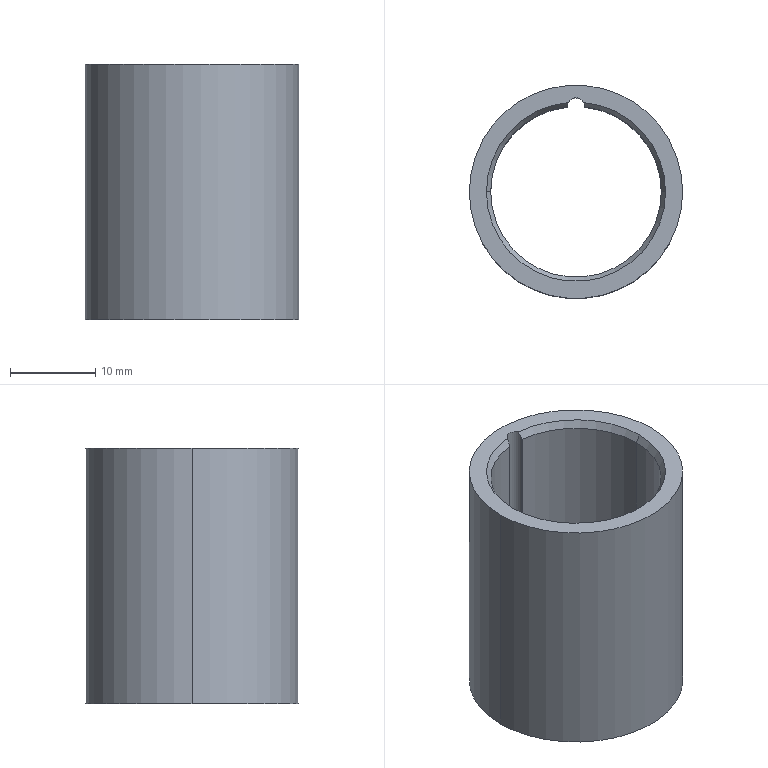Component | SolidWorks | Bushing-1 | 1 solid | 13 faces | box 25 x 25 x 30 mm | volume 5240 mm3 | cylinder 8 | cone 3 | plane 2 | commonest cylinder face diameters 2 x3 20 x3 25 x2
STEP:
#1=CARTESIAN_POINT('',(-3.217,-0.7278,5.906));
#2=VERTEX_POINT('',#1);
#3=CARTESIAN_POINT('',(-3.217,-0.7297,5.906));
#4=VERTEX_POINT('',#3);
#5=CARTESIAN_POINT('',(-3.178,-0.7278,5.906));
#6=DIRECTION('',(0.,0.,1.));
#7=DIRECTION('',(1.,0.,0.));
#8=AXIS2_PLACEMENT_3D('',#5,#6,#7);
#9=CIRCLE('',#8,0.03937);
#10=EDGE_CURVE('',#2,#4,#9,.T.);
#11=ORIENTED_EDGE('',*,*,#10,.F.);
#12=CARTESIAN_POINT('',(-3.217,-0.7278,7.056));
#13=VERTEX_POINT('',#12);
#14=CARTESIAN_POINT('',(-3.217,-0.7278,5.551));
#15=DIRECTION('',(0.,0.,1.));
#16=VECTOR('',#15,39.37);
#17=LINE('',#14,#16);
#18=EDGE_CURVE('',#2,#13,#17,.T.);
#19=ORIENTED_EDGE('',*,*,#18,.T.);
#20=CARTESIAN_POINT('',(-3.217,-0.7297,7.053));
#21=VERTEX_POINT('',#20);
#22=CARTESIAN_POINT('',(-3.217,-0.7278,7.056));
#23=CARTESIAN_POINT('',(-3.217,-0.7284,7.055));
#24=CARTESIAN_POINT('',(-3.217,-0.7291,7.054));
#25=CARTESIAN_POINT('',(-3.217,-0.7297,7.053));
#26=B_SPLINE_CURVE_WITH_KNOTS('',3,(#22,#23,#24,#25),.UNSPECIFIED.,.F.,.F.,(4,4),(0.0009137,0.001013),.UNSPECIFIED.);
#27=EDGE_CURVE('',#13,#21,#26,.T.);
#28=ORIENTED_EDGE('',*,*,#27,.T.);
#29=CARTESIAN_POINT('',(-3.217,-0.7297,7.087));
#30=DIRECTION('',(0.,0.,-1.));
#31=VECTOR('',#30,39.37);
#32=LINE('',#29,#31);
#33=EDGE_CURVE('',#21,#4,#32,.T.);
#34=ORIENTED_EDGE('',*,*,#33,.T.);
#35=EDGE_LOOP('',(#11,#19,#28,#34));
#36=FACE_OUTER_BOUND('',#35,.T.);
#37=CARTESIAN_POINT('',(-3.178,-0.7278,5.551));
#38=DIRECTION('',(0.,0.,1.));
#39=DIRECTION('',(1.,0.,0.));
#40=AXIS2_PLACEMENT_3D('',#37,#38,#39);
#41=CYLINDRICAL_SURFACE('',#40,0.03937);
#42=ADVANCED_FACE('',(#36),#41,.F.);
#43=ORIENTED_EDGE('',*,*,#18,.F.);
#44=CARTESIAN_POINT('',(-3.139,-0.7278,5.906));
#45=VERTEX_POINT('',#44);
#46=CARTESIAN_POINT('',(-3.178,-0.7278,5.906));
#47=DIRECTION('',(0.,0.,1.));
#48=DIRECTION('',(1.,0.,0.));
#49=AXIS2_PLACEMENT_3D('',#46,#47,#48);
#50=CIRCLE('',#49,0.03937);
#51=EDGE_CURVE('',#45,#2,#50,.T.);
#52=ORIENTED_EDGE('',*,*,#51,.F.);
#53=CARTESIAN_POINT('',(-3.139,-0.7278,7.056));
#54=VERTEX_POINT('',#53);
#55=CARTESIAN_POINT('',(-3.139,-0.7278,5.551));
#56=DIRECTION('',(0.,0.,1.));
#57=VECTOR('',#56,39.37);
#58=LINE('',#55,#57);
#59=EDGE_CURVE('',#45,#54,#58,.T.);
#60=ORIENTED_EDGE('',*,*,#59,.T.);
#61=CARTESIAN_POINT('',(-3.143,-0.7096,7.087));
#62=VERTEX_POINT('',#61);
#63=CARTESIAN_POINT('',(-3.139,-0.7278,7.056));
#64=CARTESIAN_POINT('',(-3.139,-0.7217,7.066));
#65=CARTESIAN_POINT('',(-3.14,-0.7156,7.077));
#66=CARTESIAN_POINT('',(-3.143,-0.7096,7.087));
#67=B_SPLINE_CURVE_WITH_KNOTS('',3,(#63,#64,#65,#66),.UNSPECIFIED.,.F.,.F.,(4,4),(0.00009929,0.001013),.UNSPECIFIED.);
#68=EDGE_CURVE('',#54,#62,#67,.T.);
#69=ORIENTED_EDGE('',*,*,#68,.T.);
#70=CARTESIAN_POINT('',(-3.213,-0.7096,7.087));
#71=VERTEX_POINT('',#70);
#72=CARTESIAN_POINT('',(-3.178,-0.7278,7.087));
#73=DIRECTION('',(0.,0.,1.));
#74=DIRECTION('',(1.,0.,0.));
#75=AXIS2_PLACEMENT_3D('',#72,#73,#74);
#76=CIRCLE('',#75,0.03937);
#77=EDGE_CURVE('',#62,#71,#76,.T.);
#78=ORIENTED_EDGE('',*,*,#77,.T.);
#79=CARTESIAN_POINT('',(-3.213,-0.7096,7.087));
#80=CARTESIAN_POINT('',(-3.216,-0.7156,7.077));
#81=CARTESIAN_POINT('',(-3.217,-0.7217,7.066));
#82=CARTESIAN_POINT('',(-3.217,-0.7278,7.056));
#83=B_SPLINE_CURVE_WITH_KNOTS('',3,(#79,#80,#81,#82),.UNSPECIFIED.,.F.,.F.,(4,4),(0.00000024,0.0009137),.UNSPECIFIED.);
#84=EDGE_CURVE('',#71,#13,#83,.T.);
#85=ORIENTED_EDGE('',*,*,#84,.T.);
#86=EDGE_LOOP('',(#43,#52,#60,#69,#78,#85));
#87=FACE_OUTER_BOUND('',#86,.T.);
#88=CARTESIAN_POINT('',(-3.178,-0.7278,5.551));
#89=DIRECTION('',(0.,0.,1.));
#90=DIRECTION('',(1.,0.,0.));
#91=AXIS2_PLACEMENT_3D('',#88,#89,#90);
#92=CYLINDRICAL_SURFACE('',#91,0.03937);
#93=ADVANCED_FACE('',(#87),#92,.F.);
#94=CARTESIAN_POINT('',(-3.572,-1.121,7.053));
#95=VERTEX_POINT('',#94);
#96=CARTESIAN_POINT('',(-2.784,-1.121,7.053));
#97=VERTEX_POINT('',#96);
#98=CARTESIAN_POINT('',(-3.178,-1.121,7.053));
#99=DIRECTION('',(0.,0.,1.));
#100=DIRECTION('',(1.,0.,0.));
#101=AXIS2_PLACEMENT_3D('',#98,#99,#100);
#102=CIRCLE('',#101,0.3937);
#103=EDGE_CURVE('',#95,#97,#102,.T.);
#104=ORIENTED_EDGE('',*,*,#103,.F.);
#105=CARTESIAN_POINT('',(-3.591,-1.121,7.087));
#106=VERTEX_POINT('',#105);
#107=CARTESIAN_POINT('',(-3.572,-1.121,7.053));
#108=DIRECTION('',(-0.5,0.,0.866));
#109=VECTOR('',#108,39.37);
#110=LINE('',#107,#109);
#111=EDGE_CURVE('',#95,#106,#110,.T.);
#112=ORIENTED_EDGE('',*,*,#111,.T.);
#113=CARTESIAN_POINT('',(-2.765,-1.121,7.087));
#114=VERTEX_POINT('',#113);
#115=CARTESIAN_POINT('',(-3.178,-1.121,7.087));
#116=DIRECTION('',(0.,0.,-1.));
#117=DIRECTION('',(1.,0.,0.));
#118=AXIS2_PLACEMENT_3D('',#115,#116,#117);
#119=CIRCLE('',#118,0.4134);
#120=EDGE_CURVE('',#114,#106,#119,.T.);
#121=ORIENTED_EDGE('',*,*,#120,.F.);
#122=CARTESIAN_POINT('',(-2.784,-1.121,7.053));
#123=DIRECTION('',(0.5,0.,0.866));
#124=VECTOR('',#123,39.37);
#125=LINE('',#122,#124);
#126=EDGE_CURVE('',#97,#114,#125,.T.);
#127=ORIENTED_EDGE('',*,*,#126,.F.);
#128=EDGE_LOOP('',(#104,#112,#121,#127));
#129=FACE_OUTER_BOUND('',#128,.T.);
#130=CARTESIAN_POINT('',(-3.178,-1.121,7.053));
#131=DIRECTION('',(0.,0.,1.));
#132=DIRECTION('',(1.,0.,0.));
#133=AXIS2_PLACEMENT_3D('',#130,#131,#132);
#134=CONICAL_SURFACE('',#133,0.3937,0.5236);
#135=ADVANCED_FACE('',(#129),#134,.F.);
#136=CARTESIAN_POINT('',(-3.139,-0.7297,7.053));
#137=VERTEX_POINT('',#136);
#138=CARTESIAN_POINT('',(-3.178,-1.121,7.053));
#139=DIRECTION('',(0.,0.,1.));
#140=DIRECTION('',(1.,0.,0.));
#141=AXIS2_PLACEMENT_3D('',#138,#139,#140);
#142=CIRCLE('',#141,0.3937);
#143=EDGE_CURVE('',#97,#137,#142,.T.);
#144=ORIENTED_EDGE('',*,*,#143,.F.);
#145=ORIENTED_EDGE('',*,*,#126,.T.);
#146=CARTESIAN_POINT('',(-3.178,-1.121,7.087));
#147=DIRECTION('',(0.,0.,-1.));
#148=DIRECTION('',(1.,-0.,0.));
#149=AXIS2_PLACEMENT_3D('',#146,#147,#148);
#150=CIRCLE('',#149,0.4134);
#151=EDGE_CURVE('',#62,#114,#150,.T.);
#152=ORIENTED_EDGE('',*,*,#151,.F.);
#153=ORIENTED_EDGE('',*,*,#68,.F.);
#154=CARTESIAN_POINT('',(-3.139,-0.7297,7.053));
#155=CARTESIAN_POINT('',(-3.139,-0.7291,7.054));
#156=CARTESIAN_POINT('',(-3.139,-0.7284,7.055));
#157=CARTESIAN_POINT('',(-3.139,-0.7278,7.056));
#158=B_SPLINE_CURVE_WITH_KNOTS('',3,(#154,#155,#156,#157),.UNSPECIFIED.,.F.,.F.,(4,4),(0.00000023,0.00009929),.UNSPECIFIED.);
#159=EDGE_CURVE('',#137,#54,#158,.T.);
#160=ORIENTED_EDGE('',*,*,#159,.F.);
#161=EDGE_LOOP('',(#144,#145,#152,#153,#160));
#162=FACE_OUTER_BOUND('',#161,.T.);
#163=CARTESIAN_POINT('',(-3.178,-1.121,7.053));
#164=DIRECTION('',(0.,0.,1.));
#165=DIRECTION('',(1.,0.,0.));
#166=AXIS2_PLACEMENT_3D('',#163,#164,#165);
#167=CONICAL_SURFACE('',#166,0.3937,0.5236);
#168=ADVANCED_FACE('',(#162),#167,.F.);
#169=ORIENTED_EDGE('',*,*,#103,.T.);
#170=CARTESIAN_POINT('',(-2.784,-1.121,5.906));
#171=VERTEX_POINT('',#170);
#172=CARTESIAN_POINT('',(-2.784,-1.121,7.087));
#173=DIRECTION('',(0.,0.,-1.));
#174=VECTOR('',#173,39.37);
#175=LINE('',#172,#174);
#176=EDGE_CURVE('',#97,#171,#175,.T.);
#177=ORIENTED_EDGE('',*,*,#176,.T.);
#178=CARTESIAN_POINT('',(-3.572,-1.121,5.906));
#179=VERTEX_POINT('',#178);
#180=CARTESIAN_POINT('',(-3.178,-1.121,5.906));
#181=DIRECTION('',(0.,0.,1.));
#182=DIRECTION('',(1.,0.,0.));
#183=AXIS2_PLACEMENT_3D('',#180,#181,#182);
#184=CIRCLE('',#183,0.3937);
#185=EDGE_CURVE('',#179,#171,#184,.T.);
#186=ORIENTED_EDGE('',*,*,#185,.F.);
#187=CARTESIAN_POINT('',(-3.572,-1.121,7.087));
#188=DIRECTION('',(0.,0.,-1.));
#189=VECTOR('',#188,39.37);
#190=LINE('',#187,#189);
#191=EDGE_CURVE('',#95,#179,#190,.T.);
#192=ORIENTED_EDGE('',*,*,#191,.F.);
#193=EDGE_LOOP('',(#169,#177,#186,#192));
#194=FACE_OUTER_BOUND('',#193,.T.);
#195=CARTESIAN_POINT('',(-3.178,-1.121,7.087));
#196=DIRECTION('',(0.,0.,-1.));
#197=DIRECTION('',(-1.,0.,0.));
#198=AXIS2_PLACEMENT_3D('',#195,#196,#197);
#199=CYLINDRICAL_SURFACE('',#198,0.3937);
#200=ADVANCED_FACE('',(#194),#199,.F.);
#201=CARTESIAN_POINT('',(-3.178,-1.121,7.053));
#202=DIRECTION('',(0.,0.,1.));
#203=DIRECTION('',(1.,0.,0.));
#204=AXIS2_PLACEMENT_3D('',#201,#202,#203);
#205=CIRCLE('',#204,0.3937);
#206=EDGE_CURVE('',#21,#95,#205,.T.);
#207=ORIENTED_EDGE('',*,*,#206,.T.);
#208=ORIENTED_EDGE('',*,*,#191,.T.);
#209=CARTESIAN_POINT('',(-3.178,-1.121,5.906));
#210=DIRECTION('',(0.,0.,1.));
#211=DIRECTION('',(1.,0.,0.));
#212=AXIS2_PLACEMENT_3D('',#209,#210,#211);
#213=CIRCLE('',#212,0.3937);
#214=EDGE_CURVE('',#4,#179,#213,.T.);
#215=ORIENTED_EDGE('',*,*,#214,.F.);
#216=ORIENTED_EDGE('',*,*,#33,.F.);
#217=EDGE_LOOP('',(#207,#208,#215,#216));
#218=FACE_OUTER_BOUND('',#217,.T.);
#219=CARTESIAN_POINT('',(-3.178,-1.121,7.087));
#220=DIRECTION('',(0.,0.,-1.));
#221=DIRECTION('',(-1.,0.,0.));
#222=AXIS2_PLACEMENT_3D('',#219,#220,#221);
#223=CYLINDRICAL_SURFACE('',#222,0.3937);
#224=ADVANCED_FACE('',(#218),#223,.F.);
#225=CARTESIAN_POINT('',(-2.686,-1.121,7.087));
#226=VERTEX_POINT('',#225);
#227=CARTESIAN_POINT('',(-3.67,-1.121,7.087));
#228=VERTEX_POINT('',#227);
#229=CARTESIAN_POINT('',(-3.178,-1.121,7.087));
#230=DIRECTION('',(0.,0.,1.));
#231=DIRECTION('',(1.,0.,0.));
#232=AXIS2_PLACEMENT_3D('',#229,#230,#231);
#233=CIRCLE('',#232,0.4921);
#234=EDGE_CURVE('',#226,#228,#233,.T.);
#235=ORIENTED_EDGE('',*,*,#234,.F.);
#236=CARTESIAN_POINT('',(-2.686,-1.121,5.906));
#237=VERTEX_POINT('',#236);
#238=CARTESIAN_POINT('',(-2.686,-1.121,7.087));
#239=DIRECTION('',(0.,0.,-1.));
#240=VECTOR('',#239,39.37);
#241=LINE('',#238,#240);
#242=EDGE_CURVE('',#226,#237,#241,.T.);
#243=ORIENTED_EDGE('',*,*,#242,.T.);
#244=CARTESIAN_POINT('',(-3.67,-1.121,5.906));
#245=VERTEX_POINT('',#244);
#246=CARTESIAN_POINT('',(-3.178,-1.121,5.906));
#247=DIRECTION('',(0.,0.,1.));
#248=DIRECTION('',(1.,0.,0.));
#249=AXIS2_PLACEMENT_3D('',#246,#247,#248);
#250=CIRCLE('',#249,0.4921);
#251=EDGE_CURVE('',#237,#245,#250,.T.);
#252=ORIENTED_EDGE('',*,*,#251,.T.);
#253=CARTESIAN_POINT('',(-3.67,-1.121,7.087));
#254=DIRECTION('',(0.,0.,-1.));
#255=VECTOR('',#254,39.37);
#256=LINE('',#253,#255);
#257=EDGE_CURVE('',#228,#245,#256,.T.);
#258=ORIENTED_EDGE('',*,*,#257,.F.);
#259=EDGE_LOOP('',(#235,#243,#252,#258));
#260=FACE_OUTER_BOUND('',#259,.T.);
#261=CARTESIAN_POINT('',(-3.178,-1.121,7.087));
#262=DIRECTION('',(0.,0.,-1.));
#263=DIRECTION('',(-1.,0.,0.));
#264=AXIS2_PLACEMENT_3D('',#261,#262,#263);
#265=CYLINDRICAL_SURFACE('',#264,0.4921);
#266=ADVANCED_FACE('',(#260),#265,.T.);
#267=ORIENTED_EDGE('',*,*,#77,.F.);
#268=ORIENTED_EDGE('',*,*,#151,.T.);
#269=ORIENTED_EDGE('',*,*,#120,.T.);
#270=CARTESIAN_POINT('',(-3.178,-1.121,7.087));
#271=DIRECTION('',(0.,0.,-1.));
#272=DIRECTION('',(1.,0.,0.));
#273=AXIS2_PLACEMENT_3D('',#270,#271,#272);
#274=CIRCLE('',#273,0.4134);
#275=EDGE_CURVE('',#106,#71,#274,.T.);
#276=ORIENTED_EDGE('',*,*,#275,.T.);
#277=EDGE_LOOP('',(#267,#268,#269,#276));
#278=FACE_BOUND('',#277,.T.);
#279=CARTESIAN_POINT('',(-3.178,-1.121,7.087));
#280=DIRECTION('',(0.,0.,1.));
#281=DIRECTION('',(1.,0.,0.));
#282=AXIS2_PLACEMENT_3D('',#279,#280,#281);
#283=CIRCLE('',#282,0.4921);
#284=EDGE_CURVE('',#228,#226,#283,.T.);
#285=ORIENTED_EDGE('',*,*,#284,.T.);
#286=ORIENTED_EDGE('',*,*,#234,.T.);
#287=EDGE_LOOP('',(#285,#286));
#288=FACE_OUTER_BOUND('',#287,.T.);
#289=CARTESIAN_POINT('',(-3.178,-1.121,7.087));
#290=DIRECTION('',(0.,0.,1.));
#291=DIRECTION('',(1.,0.,0.));
#292=AXIS2_PLACEMENT_3D('',#289,#290,#291);
#293=PLANE('',#292);
#294=ADVANCED_FACE('',(#278,#288),#293,.T.);
#295=CARTESIAN_POINT('',(-3.178,-1.121,5.906));
#296=DIRECTION('',(0.,0.,1.));
#297=DIRECTION('',(1.,0.,0.));
#298=AXIS2_PLACEMENT_3D('',#295,#296,#297);
#299=CIRCLE('',#298,0.4921);
#300=EDGE_CURVE('',#245,#237,#299,.T.);
#301=ORIENTED_EDGE('',*,*,#300,.F.);
#302=ORIENTED_EDGE('',*,*,#251,.F.);
#303=EDGE_LOOP('',(#301,#302));
#304=FACE_OUTER_BOUND('',#303,.T.);
#305=ORIENTED_EDGE('',*,*,#214,.T.);
#306=ORIENTED_EDGE('',*,*,#185,.T.);
#307=CARTESIAN_POINT('',(-3.139,-0.7297,5.906));
#308=VERTEX_POINT('',#307);
#309=CARTESIAN_POINT('',(-3.178,-1.121,5.906));
#310=DIRECTION('',(0.,0.,1.));
#311=DIRECTION('',(1.,0.,0.));
#312=AXIS2_PLACEMENT_3D('',#309,#310,#311);
#313=CIRCLE('',#312,0.3937);
#314=EDGE_CURVE('',#171,#308,#313,.T.);
#315=ORIENTED_EDGE('',*,*,#314,.T.);
#316=CARTESIAN_POINT('',(-3.178,-0.7278,5.906));
#317=DIRECTION('',(0.,0.,1.));
#318=DIRECTION('',(1.,0.,0.));
#319=AXIS2_PLACEMENT_3D('',#316,#317,#318);
#320=CIRCLE('',#319,0.03937);
#321=EDGE_CURVE('',#308,#45,#320,.T.);
#322=ORIENTED_EDGE('',*,*,#321,.T.);
#323=ORIENTED_EDGE('',*,*,#51,.T.);
#324=ORIENTED_EDGE('',*,*,#10,.T.);
#325=EDGE_LOOP('',(#305,#306,#315,#322,#323,#324));
#326=FACE_BOUND('',#325,.T.);
#327=CARTESIAN_POINT('',(-3.178,-1.121,5.906));
#328=DIRECTION('',(0.,0.,1.));
#329=DIRECTION('',(1.,0.,0.));
#330=AXIS2_PLACEMENT_3D('',#327,#328,#329);
#331=PLANE('',#330);
#332=ADVANCED_FACE('',(#304,#326),#331,.F.);
#333=ORIENTED_EDGE('',*,*,#242,.F.);
#334=ORIENTED_EDGE('',*,*,#284,.F.);
#335=ORIENTED_EDGE('',*,*,#257,.T.);
#336=ORIENTED_EDGE('',*,*,#300,.T.);
#337=EDGE_LOOP('',(#333,#334,#335,#336));
#338=FACE_OUTER_BOUND('',#337,.T.);
#339=CARTESIAN_POINT('',(-3.178,-1.121,7.087));
#340=DIRECTION('',(0.,0.,-1.));
#341=DIRECTION('',(-1.,0.,0.));
#342=AXIS2_PLACEMENT_3D('',#339,#340,#341);
#343=CYLINDRICAL_SURFACE('',#342,0.4921);
#344=ADVANCED_FACE('',(#338),#343,.T.);
#345=ORIENTED_EDGE('',*,*,#176,.F.);
#346=ORIENTED_EDGE('',*,*,#143,.T.);
#347=CARTESIAN_POINT('',(-3.139,-0.7297,7.087));
#348=DIRECTION('',(0.,0.,1.));
#349=VECTOR('',#348,39.37);
#350=LINE('',#347,#349);
#351=EDGE_CURVE('',#308,#137,#350,.T.);
#352=ORIENTED_EDGE('',*,*,#351,.F.);
#353=ORIENTED_EDGE('',*,*,#314,.F.);
#354=EDGE_LOOP('',(#345,#346,#352,#353));
#355=FACE_OUTER_BOUND('',#354,.T.);
#356=CARTESIAN_POINT('',(-3.178,-1.121,7.087));
#357=DIRECTION('',(0.,0.,-1.));
#358=DIRECTION('',(-1.,0.,0.));
#359=AXIS2_PLACEMENT_3D('',#356,#357,#358);
#360=CYLINDRICAL_SURFACE('',#359,0.3937);
#361=ADVANCED_FACE('',(#355),#360,.F.);
#362=ORIENTED_EDGE('',*,*,#111,.F.);
#363=ORIENTED_EDGE('',*,*,#206,.F.);
#364=ORIENTED_EDGE('',*,*,#27,.F.);
#365=ORIENTED_EDGE('',*,*,#84,.F.);
#366=ORIENTED_EDGE('',*,*,#275,.F.);
#367=EDGE_LOOP('',(#362,#363,#364,#365,#366));
#368=FACE_OUTER_BOUND('',#367,.T.);
#369=CARTESIAN_POINT('',(-3.178,-1.121,7.053));
#370=DIRECTION('',(0.,0.,1.));
#371=DIRECTION('',(1.,0.,0.));
#372=AXIS2_PLACEMENT_3D('',#369,#370,#371);
#373=CONICAL_SURFACE('',#372,0.3937,0.5236);
#374=ADVANCED_FACE('',(#368),#373,.F.);
#375=ORIENTED_EDGE('',*,*,#59,.F.);
#376=ORIENTED_EDGE('',*,*,#321,.F.);
#377=ORIENTED_EDGE('',*,*,#351,.T.);
#378=ORIENTED_EDGE('',*,*,#159,.T.);
#379=EDGE_LOOP('',(#375,#376,#377,#378));
#380=FACE_OUTER_BOUND('',#379,.T.);
#381=CARTESIAN_POINT('',(-3.178,-0.7278,5.551));
#382=DIRECTION('',(0.,0.,1.));
#383=DIRECTION('',(1.,0.,0.));
#384=AXIS2_PLACEMENT_3D('',#381,#382,#383);
#385=CYLINDRICAL_SURFACE('',#384,0.03937);
#386=ADVANCED_FACE('',(#380),#385,.F.);
#387=CLOSED_SHELL('',(#42,#93,#135,#168,#200,#224,#266,#294,#332,#344,#361,#374,#386));
#388=MANIFOLD_SOLID_BREP('',#387);
#389=CARTESIAN_POINT('',(0.,0.,0.));
#390=DIRECTION('',(0.,0.,1.));
#391=DIRECTION('',(1.,0.,0.));
#392=AXIS2_PLACEMENT_3D('',#389,#390,#391);
#393=(LENGTH_UNIT()NAMED_UNIT(*)SI_UNIT($,.METRE.));
#394=LENGTH_MEASURE_WITH_UNIT(LENGTH_MEASURE(0.0254),#393);
#395=DIMENSIONAL_EXPONENTS(1.,0.,0.,0.,0.,0.,0.);
#396=(CONVERSION_BASED_UNIT('',#394)LENGTH_UNIT()NAMED_UNIT(#395));
#397=UNCERTAINTY_MEASURE_WITH_UNIT(LENGTH_MEASURE(0.00001),#396,'','');
#398=(NAMED_UNIT(*)PLANE_ANGLE_UNIT()SI_UNIT($,.RADIAN.));
#399=(NAMED_UNIT(*)SI_UNIT($,.STERADIAN.)SOLID_ANGLE_UNIT());
#400=(GEOMETRIC_REPRESENTATION_CONTEXT(3)GLOBAL_UNCERTAINTY_ASSIGNED_CONTEXT((#397))GLOBAL_UNIT_ASSIGNED_CONTEXT((#396,#398,#399))REPRESENTATION_CONTEXT('',''));
#401=ADVANCED_BREP_SHAPE_REPRESENTATION('',(#388,#392),#400);
#402=COLOUR_RGB('',0.7922,0.8196,0.9333);
#403=FILL_AREA_STYLE_COLOUR('',#402);
#404=FILL_AREA_STYLE('',(#403));
#405=SURFACE_STYLE_FILL_AREA(#404);
#406=SURFACE_SIDE_STYLE('',(#405));
#407=SURFACE_STYLE_USAGE(.BOTH.,#406);
#408=PRESENTATION_STYLE_ASSIGNMENT((#407));
#409=STYLED_ITEM('',(#408),#388);
#410=(LENGTH_UNIT()NAMED_UNIT(*)SI_UNIT($,.METRE.));
#411=LENGTH_MEASURE_WITH_UNIT(LENGTH_MEASURE(0.0254),#410);
#412=DIMENSIONAL_EXPONENTS(1.,0.,0.,0.,0.,0.,0.);
#413=(CONVERSION_BASED_UNIT('',#411)LENGTH_UNIT()NAMED_UNIT(#412));
#414=UNCERTAINTY_MEASURE_WITH_UNIT(LENGTH_MEASURE(0.00001),#413,'','');
#415=(NAMED_UNIT(*)PLANE_ANGLE_UNIT()SI_UNIT($,.RADIAN.));
#416=(NAMED_UNIT(*)SI_UNIT($,.STERADIAN.)SOLID_ANGLE_UNIT());
#417=(GEOMETRIC_REPRESENTATION_CONTEXT(3)GLOBAL_UNCERTAINTY_ASSIGNED_CONTEXT((#414))GLOBAL_UNIT_ASSIGNED_CONTEXT((#413,#415,#416))REPRESENTATION_CONTEXT('',''));
#418=MECHANICAL_DESIGN_GEOMETRIC_PRESENTATION_REPRESENTATION('',(#409),#417);
#419=PRESENTATION_LAYER_ASSIGNMENT('','',(#409));